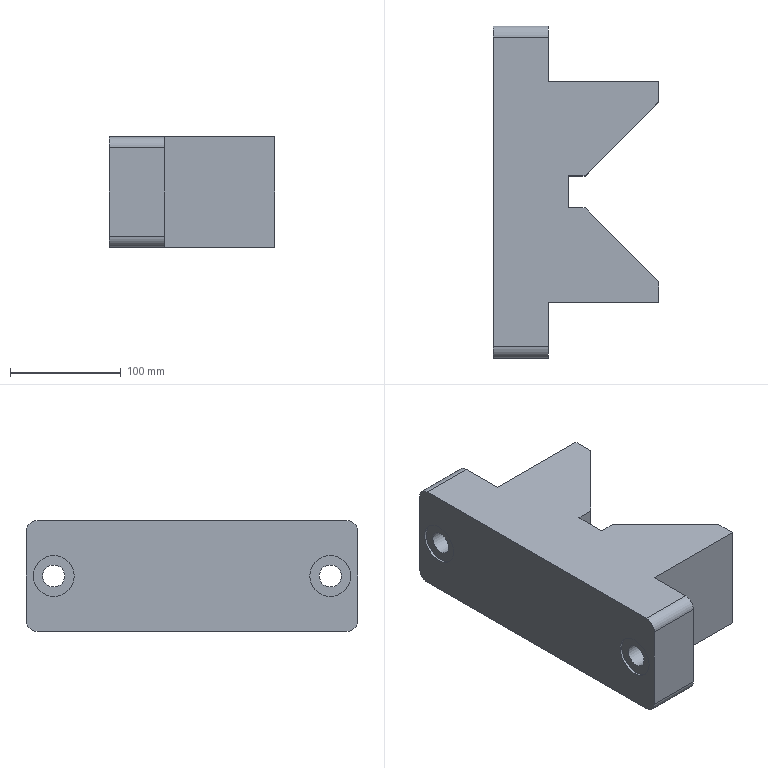Component | NX | V_BLOCK | 1 solid | 26 faces | volume 2777521 mm3 | plane 18 | cylinder 8 | commonest cylinder face diameters 20 x6 37 x2